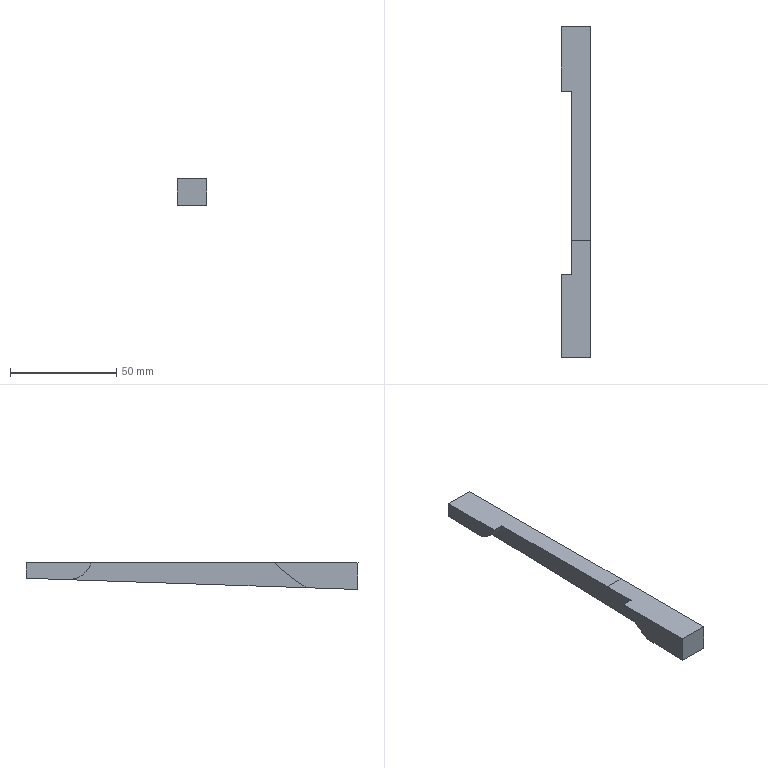Component | NX | UPPER_WEDGE | 1 solid | 11 faces | box 14 x 156.34 x 12.64 mm | volume 17054 mm3 | plane 9 | cylinder 2 | commonest cylinder face diameters 22.759 x1 150 x1
STEP:
#1=CARTESIAN_POINT('',(0.,0.,0.));
#2=DIRECTION('',(0.,0.,1.));
#3=DIRECTION('',(1.,0.,0.));
#4=AXIS2_PLACEMENT_3D('',#1,#2,#3);
#5=CARTESIAN_POINT('',(-109.,42.593,69.43));
#6=VERTEX_POINT('',#5);
#7=CARTESIAN_POINT('',(-109.,53.838,61.449));
#8=VERTEX_POINT('',#7);
#9=CARTESIAN_POINT('',(-109.,53.456,72.821));
#10=DIRECTION('',(1.,0.,0.));
#11=DIRECTION('',(0.,1.,-0.0009895));
#12=AXIS2_PLACEMENT_3D('',#9,#10,#11);
#13=CIRCLE('',#12,11.379);
#14=CARTESIAN_POINT('',(-109.,73.093,69.4));
#15=DIRECTION('',(-1.,0.,0.));
#16=DIRECTION('',(0.,0.03361,-0.9994));
#17=AXIS2_PLACEMENT_3D('',#14,#15,#16);
#18=PLANE('',#17);
#19=CARTESIAN_POINT('',(-3.686,8.139));
#20=CARTESIAN_POINT('',(-23.383,7.457));
#21=CARTESIAN_POINT('',(-14.125,24.857));
#22=CARTESIAN_POINT('',(-4.867,42.257));
#23=CARTESIAN_POINT('',(5.573,25.539));
#24=CARTESIAN_POINT('',(16.012,8.821));
#25=CARTESIAN_POINT('',(-3.686,8.139));
#26=(BOUNDED_CURVE()B_SPLINE_CURVE(2,(#19,#20,#21,#22,#23,#24,#25),.UNSPECIFIED.,.T.,.F.)B_SPLINE_CURVE_WITH_KNOTS((1,2,2,2,2,1),(-2.094,0.,2.094,4.189,6.283,8.378),.UNSPECIFIED.)CURVE()GEOMETRIC_REPRESENTATION_ITEM()RATIONAL_B_SPLINE_CURVE((1.,0.5,1.,0.5,1.,0.5,1.))REPRESENTATION_ITEM(''));
#27=(GEOMETRIC_REPRESENTATION_CONTEXT(2)PARAMETRIC_REPRESENTATION_CONTEXT()REPRESENTATION_CONTEXT('',''));
#28=DEFINITIONAL_REPRESENTATION('',(#26),#27);
#29=PCURVE('',#18,#28);
#30=CARTESIAN_POINT('',(-104.,53.456,72.821));
#31=DIRECTION('',(-1.,0.,0.));
#32=DIRECTION('',(0.,0.03361,-0.9994));
#33=AXIS2_PLACEMENT_3D('',#30,#31,#32);
#34=CYLINDRICAL_SURFACE('',#33,11.379);
#35=CARTESIAN_POINT('',(4.747,5.));
#36=DIRECTION('',(-1.,0.));
#37=VECTOR('',#36,1.);
#38=LINE('',#35,#37);
#39=(GEOMETRIC_REPRESENTATION_CONTEXT(2)PARAMETRIC_REPRESENTATION_CONTEXT()REPRESENTATION_CONTEXT('',''));
#40=DEFINITIONAL_REPRESENTATION('',(#38),#39);
#41=PCURVE('',#34,#40);
#42=SURFACE_CURVE('',#13,(#29,#41),.PCURVE_S1.);
#43=EDGE_CURVE('',#6,#8,#42,.T.);
#44=ORIENTED_EDGE('',*,*,#43,.F.);
#45=CARTESIAN_POINT('',(-109.,73.093,69.4));
#46=VERTEX_POINT('',#45);
#47=CARTESIAN_POINT('',(-109.,-83.,69.555));
#48=DIRECTION('',(0.,1.,-0.0009895));
#49=VECTOR('',#48,1.);
#50=LINE('',#47,#49);
#51=CARTESIAN_POINT('',(-5.4,156.));
#52=DIRECTION('',(0.03459,-0.9994));
#53=VECTOR('',#52,1.);
#54=LINE('',#51,#53);
#55=(GEOMETRIC_REPRESENTATION_CONTEXT(2)PARAMETRIC_REPRESENTATION_CONTEXT()REPRESENTATION_CONTEXT('',''));
#56=DEFINITIONAL_REPRESENTATION('',(#54),#55);
#57=PCURVE('',#18,#56);
#58=CARTESIAN_POINT('',(-95.,73.093,69.4));
#59=DIRECTION('',(0.,-0.0009895,-1.));
#60=DIRECTION('',(0.,1.,-0.0009895));
#61=AXIS2_PLACEMENT_3D('',#58,#59,#60);
#62=PLANE('',#61);
#63=CARTESIAN_POINT('',(-156.093,-14.));
#64=DIRECTION('',(1.,0.));
#65=VECTOR('',#64,1.);
#66=LINE('',#63,#65);
#67=(GEOMETRIC_REPRESENTATION_CONTEXT(2)PARAMETRIC_REPRESENTATION_CONTEXT()REPRESENTATION_CONTEXT('',''));
#68=DEFINITIONAL_REPRESENTATION('',(#66),#67);
#69=PCURVE('',#62,#68);
#70=SURFACE_CURVE('',#50,(#57,#69),.PCURVE_S1.);
#71=EDGE_CURVE('',#6,#46,#70,.T.);
#72=ORIENTED_EDGE('',*,*,#71,.T.);
#73=CARTESIAN_POINT('',(-109.,73.339,62.104));
#74=VERTEX_POINT('',#73);
#75=CARTESIAN_POINT('',(-109.,73.093,69.4));
#76=DIRECTION('',(0.,0.03361,-0.9994));
#77=VECTOR('',#76,1.);
#78=LINE('',#75,#77);
#79=CARTESIAN_POINT('',(0.,0.));
#80=DIRECTION('',(1.,0.));
#81=VECTOR('',#80,1.);
#82=LINE('',#79,#81);
#83=(GEOMETRIC_REPRESENTATION_CONTEXT(2)PARAMETRIC_REPRESENTATION_CONTEXT()REPRESENTATION_CONTEXT('',''));
#84=DEFINITIONAL_REPRESENTATION('',(#82),#83);
#85=PCURVE('',#18,#84);
#86=CARTESIAN_POINT('',(-95.,73.339,62.104));
#87=DIRECTION('',(0.,-0.9994,-0.03361));
#88=DIRECTION('',(0.,0.03361,-0.9994));
#89=AXIS2_PLACEMENT_3D('',#86,#87,#88);
#90=PLANE('',#89);
#91=CARTESIAN_POINT('',(-7.3,-14.));
#92=DIRECTION('',(1.,0.));
#93=VECTOR('',#92,1.);
#94=LINE('',#91,#93);
#95=(GEOMETRIC_REPRESENTATION_CONTEXT(2)PARAMETRIC_REPRESENTATION_CONTEXT()REPRESENTATION_CONTEXT('',''));
#96=DEFINITIONAL_REPRESENTATION('',(#94),#95);
#97=PCURVE('',#90,#96);
#98=SURFACE_CURVE('',#78,(#85,#97),.PCURVE_S1.);
#99=EDGE_CURVE('',#46,#74,#98,.T.);
#100=ORIENTED_EDGE('',*,*,#99,.T.);
#101=CARTESIAN_POINT('',(-109.,73.339,62.104));
#102=DIRECTION('',(0.,-0.9994,-0.03361));
#103=VECTOR('',#102,1.);
#104=LINE('',#101,#103);
#105=CARTESIAN_POINT('',(7.3,-0.));
#106=DIRECTION('',(-0.,1.));
#107=VECTOR('',#106,1.);
#108=LINE('',#105,#107);
#109=(GEOMETRIC_REPRESENTATION_CONTEXT(2)PARAMETRIC_REPRESENTATION_CONTEXT()REPRESENTATION_CONTEXT('',''));
#110=DEFINITIONAL_REPRESENTATION('',(#108),#109);
#111=PCURVE('',#18,#110);
#112=CARTESIAN_POINT('',(-95.,-82.573,56.862));
#113=DIRECTION('',(0.,-0.03361,0.9994));
#114=DIRECTION('',(-1.,0.,0.));
#115=AXIS2_PLACEMENT_3D('',#112,#113,#114);
#116=PLANE('',#115);
#117=CARTESIAN_POINT('',(14.,-156.));
#118=DIRECTION('',(0.,1.));
#119=VECTOR('',#118,1.);
#120=LINE('',#117,#119);
#121=(GEOMETRIC_REPRESENTATION_CONTEXT(2)PARAMETRIC_REPRESENTATION_CONTEXT()REPRESENTATION_CONTEXT('',''));
#122=DEFINITIONAL_REPRESENTATION('',(#120),#121);
#123=PCURVE('',#116,#122);
#124=SURFACE_CURVE('',#104,(#111,#123),.PCURVE_S1.);
#125=EDGE_CURVE('',#74,#8,#124,.T.);
#126=ORIENTED_EDGE('',*,*,#125,.T.);
#127=EDGE_LOOP('',(#44,#72,#100,#126));
#128=FACE_BOUND('',#127,.T.);
#129=ADVANCED_FACE('',(#128),#18,.T.);
#130=CARTESIAN_POINT('',(-109.,-43.516,69.5));
#131=VERTEX_POINT('',#130);
#132=CARTESIAN_POINT('',(-109.,-82.998,69.5));
#133=VERTEX_POINT('',#132);
#134=CARTESIAN_POINT('',(-109.,73.093,69.5));
#135=DIRECTION('',(0.,-1.,0.));
#136=VECTOR('',#135,1.);
#137=LINE('',#134,#136);
#138=CARTESIAN_POINT('',(-109.,73.093,69.4));
#139=DIRECTION('',(-1.,0.,0.));
#140=DIRECTION('',(0.,0.03361,-0.9994));
#141=AXIS2_PLACEMENT_3D('',#138,#139,#140);
#142=PLANE('',#141);
#143=CARTESIAN_POINT('',(-0.09982,-0.003356));
#144=DIRECTION('',(-0.03361,0.9994));
#145=VECTOR('',#144,1.);
#146=LINE('',#143,#145);
#147=(GEOMETRIC_REPRESENTATION_CONTEXT(2)PARAMETRIC_REPRESENTATION_CONTEXT()REPRESENTATION_CONTEXT('',''));
#148=DEFINITIONAL_REPRESENTATION('',(#146),#147);
#149=PCURVE('',#142,#148);
#150=CARTESIAN_POINT('',(-100.,0.,69.5));
#151=DIRECTION('',(0.,0.,-1.));
#152=DIRECTION('',(-1.,0.,0.));
#153=AXIS2_PLACEMENT_3D('',#150,#151,#152);
#154=PLANE('',#153);
#155=CARTESIAN_POINT('',(9.,73.093));
#156=DIRECTION('',(0.,-1.));
#157=VECTOR('',#156,1.);
#158=LINE('',#155,#157);
#159=(GEOMETRIC_REPRESENTATION_CONTEXT(2)PARAMETRIC_REPRESENTATION_CONTEXT()REPRESENTATION_CONTEXT('',''));
#160=DEFINITIONAL_REPRESENTATION('',(#158),#159);
#161=PCURVE('',#154,#160);
#162=SURFACE_CURVE('',#137,(#149,#161),.PCURVE_S1.);
#163=EDGE_CURVE('',#131,#133,#162,.T.);
#164=ORIENTED_EDGE('',*,*,#163,.F.);
#165=CARTESIAN_POINT('',(-109.,-59.072,57.652));
#166=VERTEX_POINT('',#165);
#167=CARTESIAN_POINT('',(-109.,-96.348,122.733));
#168=DIRECTION('',(1.,0.,0.));
#169=DIRECTION('',(0.,1.,-0.0009895));
#170=AXIS2_PLACEMENT_3D('',#167,#168,#169);
#171=CIRCLE('',#170,75.);
#172=CARTESIAN_POINT('',(-56.402,92.598));
#173=CARTESIAN_POINT('',(-186.228,88.104));
#174=CARTESIAN_POINT('',(-125.207,202.784));
#175=CARTESIAN_POINT('',(-64.186,317.464));
#176=CARTESIAN_POINT('',(4.619,207.278));
#177=CARTESIAN_POINT('',(73.424,97.092));
#178=CARTESIAN_POINT('',(-56.402,92.598));
#179=(BOUNDED_CURVE()B_SPLINE_CURVE(2,(#172,#173,#174,#175,#176,#177,#178),.UNSPECIFIED.,.T.,.F.)B_SPLINE_CURVE_WITH_KNOTS((1,2,2,2,2,1),(-2.094,0.,2.094,4.189,6.283,8.378),.UNSPECIFIED.)CURVE()GEOMETRIC_REPRESENTATION_ITEM()RATIONAL_B_SPLINE_CURVE((1.,0.5,1.,0.5,1.,0.5,1.))REPRESENTATION_ITEM(''));
#180=(GEOMETRIC_REPRESENTATION_CONTEXT(2)PARAMETRIC_REPRESENTATION_CONTEXT()REPRESENTATION_CONTEXT('',''));
#181=DEFINITIONAL_REPRESENTATION('',(#179),#180);
#182=PCURVE('',#142,#181);
#183=CARTESIAN_POINT('',(-104.,-96.348,122.733));
#184=DIRECTION('',(-1.,0.,0.));
#185=DIRECTION('',(0.,0.03361,-0.9994));
#186=AXIS2_PLACEMENT_3D('',#183,#184,#185);
#187=CYLINDRICAL_SURFACE('',#186,75.);
#188=CARTESIAN_POINT('',(11.03,5.));
#189=DIRECTION('',(-1.,0.));
#190=VECTOR('',#189,1.);
#191=LINE('',#188,#190);
#192=(GEOMETRIC_REPRESENTATION_CONTEXT(2)PARAMETRIC_REPRESENTATION_CONTEXT()REPRESENTATION_CONTEXT('',''));
#193=DEFINITIONAL_REPRESENTATION('',(#191),#192);
#194=PCURVE('',#187,#193);
#195=SURFACE_CURVE('',#171,(#182,#194),.PCURVE_S1.);
#196=EDGE_CURVE('',#166,#131,#195,.T.);
#197=ORIENTED_EDGE('',*,*,#196,.F.);
#198=CARTESIAN_POINT('',(-109.,-82.573,56.862));
#199=VERTEX_POINT('',#198);
#200=CARTESIAN_POINT('',(-109.,73.339,62.104));
#201=DIRECTION('',(0.,-0.9994,-0.03361));
#202=VECTOR('',#201,1.);
#203=LINE('',#200,#202);
#204=CARTESIAN_POINT('',(7.3,-0.));
#205=DIRECTION('',(-0.,1.));
#206=VECTOR('',#205,1.);
#207=LINE('',#204,#206);
#208=(GEOMETRIC_REPRESENTATION_CONTEXT(2)PARAMETRIC_REPRESENTATION_CONTEXT()REPRESENTATION_CONTEXT('',''));
#209=DEFINITIONAL_REPRESENTATION('',(#207),#208);
#210=PCURVE('',#142,#209);
#211=CARTESIAN_POINT('',(14.,-156.));
#212=DIRECTION('',(0.,1.));
#213=VECTOR('',#212,1.);
#214=LINE('',#211,#213);
#215=(GEOMETRIC_REPRESENTATION_CONTEXT(2)PARAMETRIC_REPRESENTATION_CONTEXT()REPRESENTATION_CONTEXT('',''));
#216=DEFINITIONAL_REPRESENTATION('',(#214),#215);
#217=PCURVE('',#116,#216);
#218=SURFACE_CURVE('',#203,(#210,#217),.PCURVE_S1.);
#219=EDGE_CURVE('',#166,#199,#218,.T.);
#220=ORIENTED_EDGE('',*,*,#219,.T.);
#221=CARTESIAN_POINT('',(-109.,-82.573,56.862));
#222=DIRECTION('',(0.,-0.03361,0.9994));
#223=VECTOR('',#222,1.);
#224=LINE('',#221,#223);
#225=CARTESIAN_POINT('',(7.3,156.));
#226=DIRECTION('',(-1.,0.));
#227=VECTOR('',#226,1.);
#228=LINE('',#225,#227);
#229=(GEOMETRIC_REPRESENTATION_CONTEXT(2)PARAMETRIC_REPRESENTATION_CONTEXT()REPRESENTATION_CONTEXT('',''));
#230=DEFINITIONAL_REPRESENTATION('',(#228),#229);
#231=PCURVE('',#142,#230);
#232=CARTESIAN_POINT('',(-95.,-83.,69.555));
#233=DIRECTION('',(0.,0.9994,0.03361));
#234=DIRECTION('',(0.,-0.03361,0.9994));
#235=AXIS2_PLACEMENT_3D('',#232,#233,#234);
#236=PLANE('',#235);
#237=CARTESIAN_POINT('',(-12.7,-14.));
#238=DIRECTION('',(1.,0.));
#239=VECTOR('',#238,1.);
#240=LINE('',#237,#239);
#241=(GEOMETRIC_REPRESENTATION_CONTEXT(2)PARAMETRIC_REPRESENTATION_CONTEXT()REPRESENTATION_CONTEXT('',''));
#242=DEFINITIONAL_REPRESENTATION('',(#240),#241);
#243=PCURVE('',#236,#242);
#244=SURFACE_CURVE('',#224,(#231,#243),.PCURVE_S1.);
#245=EDGE_CURVE('',#199,#133,#244,.T.);
#246=ORIENTED_EDGE('',*,*,#245,.T.);
#247=EDGE_LOOP('',(#164,#197,#220,#246));
#248=FACE_BOUND('',#247,.T.);
#249=ADVANCED_FACE('',(#248),#142,.T.);
#250=ORIENTED_EDGE('',*,*,#99,.F.);
#251=CARTESIAN_POINT('',(-95.,73.093,69.4));
#252=VERTEX_POINT('',#251);
#253=CARTESIAN_POINT('',(-95.,73.093,69.4));
#254=DIRECTION('',(-1.,0.,0.));
#255=VECTOR('',#254,1.);
#256=LINE('',#253,#255);
#257=CARTESIAN_POINT('',(-7.3,0.));
#258=DIRECTION('',(0.,-1.));
#259=VECTOR('',#258,1.);
#260=LINE('',#257,#259);
#261=(GEOMETRIC_REPRESENTATION_CONTEXT(2)PARAMETRIC_REPRESENTATION_CONTEXT()REPRESENTATION_CONTEXT('',''));
#262=DEFINITIONAL_REPRESENTATION('',(#260),#261);
#263=PCURVE('',#90,#262);
#264=CARTESIAN_POINT('',(0.,0.));
#265=DIRECTION('',(0.,-1.));
#266=VECTOR('',#265,1.);
#267=LINE('',#264,#266);
#268=(GEOMETRIC_REPRESENTATION_CONTEXT(2)PARAMETRIC_REPRESENTATION_CONTEXT()REPRESENTATION_CONTEXT('',''));
#269=DEFINITIONAL_REPRESENTATION('',(#267),#268);
#270=PCURVE('',#62,#269);
#271=SURFACE_CURVE('',#256,(#263,#270),.PCURVE_S1.);
#272=EDGE_CURVE('',#252,#46,#271,.T.);
#273=ORIENTED_EDGE('',*,*,#272,.F.);
#274=CARTESIAN_POINT('',(-95.,73.339,62.104));
#275=VERTEX_POINT('',#274);
#276=CARTESIAN_POINT('',(-95.,73.339,62.104));
#277=DIRECTION('',(0.,-0.03361,0.9994));
#278=VECTOR('',#277,1.);
#279=LINE('',#276,#278);
#280=CARTESIAN_POINT('',(0.,0.));
#281=DIRECTION('',(-1.,0.));
#282=VECTOR('',#281,1.);
#283=LINE('',#280,#282);
#284=(GEOMETRIC_REPRESENTATION_CONTEXT(2)PARAMETRIC_REPRESENTATION_CONTEXT()REPRESENTATION_CONTEXT('',''));
#285=DEFINITIONAL_REPRESENTATION('',(#283),#284);
#286=PCURVE('',#90,#285);
#287=CARTESIAN_POINT('',(-95.,73.093,69.4));
#288=DIRECTION('',(-1.,0.,0.));
#289=DIRECTION('',(0.,0.03361,-0.9994));
#290=AXIS2_PLACEMENT_3D('',#287,#288,#289);
#291=PLANE('',#290);
#292=CARTESIAN_POINT('',(7.3,-0.));
#293=DIRECTION('',(-1.,0.));
#294=VECTOR('',#293,1.);
#295=LINE('',#292,#294);
#296=(GEOMETRIC_REPRESENTATION_CONTEXT(2)PARAMETRIC_REPRESENTATION_CONTEXT()REPRESENTATION_CONTEXT('',''));
#297=DEFINITIONAL_REPRESENTATION('',(#295),#296);
#298=PCURVE('',#291,#297);
#299=SURFACE_CURVE('',#279,(#286,#298),.PCURVE_S1.);
#300=EDGE_CURVE('',#275,#252,#299,.T.);
#301=ORIENTED_EDGE('',*,*,#300,.F.);
#302=CARTESIAN_POINT('',(-95.,73.339,62.104));
#303=DIRECTION('',(-1.,0.,0.));
#304=VECTOR('',#303,1.);
#305=LINE('',#302,#304);
#306=CARTESIAN_POINT('',(0.,0.));
#307=DIRECTION('',(0.,-1.));
#308=VECTOR('',#307,1.);
#309=LINE('',#306,#308);
#310=(GEOMETRIC_REPRESENTATION_CONTEXT(2)PARAMETRIC_REPRESENTATION_CONTEXT()REPRESENTATION_CONTEXT('',''));
#311=DEFINITIONAL_REPRESENTATION('',(#309),#310);
#312=PCURVE('',#90,#311);
#313=CARTESIAN_POINT('',(0.,-156.));
#314=DIRECTION('',(1.,0.));
#315=VECTOR('',#314,1.);
#316=LINE('',#313,#315);
#317=(GEOMETRIC_REPRESENTATION_CONTEXT(2)PARAMETRIC_REPRESENTATION_CONTEXT()REPRESENTATION_CONTEXT('',''));
#318=DEFINITIONAL_REPRESENTATION('',(#316),#317);
#319=PCURVE('',#116,#318);
#320=SURFACE_CURVE('',#305,(#312,#319),.PCURVE_S1.);
#321=EDGE_CURVE('',#275,#74,#320,.T.);
#322=ORIENTED_EDGE('',*,*,#321,.T.);
#323=EDGE_LOOP('',(#250,#273,#301,#322));
#324=FACE_BOUND('',#323,.T.);
#325=ADVANCED_FACE('',(#324),#90,.F.);
#326=CARTESIAN_POINT('',(-104.,-27.834,69.5));
#327=VERTEX_POINT('',#326);
#328=CARTESIAN_POINT('',(-104.,42.593,69.43));
#329=VERTEX_POINT('',#328);
#330=CARTESIAN_POINT('',(-104.,-43.5,69.516));
#331=DIRECTION('',(0.,1.,-0.0009895));
#332=VECTOR('',#331,1.);
#333=LINE('',#330,#332);
#334=CARTESIAN_POINT('',(-116.593,-9.));
#335=DIRECTION('',(1.,0.));
#336=VECTOR('',#335,1.);
#337=LINE('',#334,#336);
#338=(GEOMETRIC_REPRESENTATION_CONTEXT(2)PARAMETRIC_REPRESENTATION_CONTEXT()REPRESENTATION_CONTEXT('',''));
#339=DEFINITIONAL_REPRESENTATION('',(#337),#338);
#340=PCURVE('',#62,#339);
#341=CARTESIAN_POINT('',(-104.,53.456,72.821));
#342=DIRECTION('',(1.,0.,0.));
#343=DIRECTION('',(0.,-0.03361,0.9994));
#344=AXIS2_PLACEMENT_3D('',#341,#342,#343);
#345=PLANE('',#344);
#346=CARTESIAN_POINT('',(-0.04575,97.012));
#347=DIRECTION('',(-0.03459,-0.9994));
#348=VECTOR('',#347,1.);
#349=LINE('',#346,#348);
#350=(GEOMETRIC_REPRESENTATION_CONTEXT(2)PARAMETRIC_REPRESENTATION_CONTEXT()REPRESENTATION_CONTEXT('',''));
#351=DEFINITIONAL_REPRESENTATION('',(#349),#350);
#352=PCURVE('',#345,#351);
#353=SURFACE_CURVE('',#333,(#340,#352),.PCURVE_S1.);
#354=EDGE_CURVE('',#327,#329,#353,.T.);
#355=ORIENTED_EDGE('',*,*,#354,.F.);
#356=CARTESIAN_POINT('',(-95.,-27.834,69.5));
#357=VERTEX_POINT('',#356);
#358=CARTESIAN_POINT('',(-95.,-27.834,69.5));
#359=DIRECTION('',(1.,0.,0.));
#360=VECTOR('',#359,1.);
#361=LINE('',#358,#360);
#362=CARTESIAN_POINT('',(-100.928,0.));
#363=DIRECTION('',(0.,1.));
#364=VECTOR('',#363,1.);
#365=LINE('',#362,#364);
#366=(GEOMETRIC_REPRESENTATION_CONTEXT(2)PARAMETRIC_REPRESENTATION_CONTEXT()REPRESENTATION_CONTEXT('',''));
#367=DEFINITIONAL_REPRESENTATION('',(#365),#366);
#368=PCURVE('',#62,#367);
#369=CARTESIAN_POINT('',(-5.,-27.834));
#370=DIRECTION('',(-1.,0.));
#371=VECTOR('',#370,1.);
#372=LINE('',#369,#371);
#373=(GEOMETRIC_REPRESENTATION_CONTEXT(2)PARAMETRIC_REPRESENTATION_CONTEXT()REPRESENTATION_CONTEXT('',''));
#374=DEFINITIONAL_REPRESENTATION('',(#372),#373);
#375=PCURVE('',#154,#374);
#376=SURFACE_CURVE('',#361,(#368,#375),.PCURVE_S1.);
#377=EDGE_CURVE('',#327,#357,#376,.T.);
#378=ORIENTED_EDGE('',*,*,#377,.T.);
#379=CARTESIAN_POINT('',(-95.,73.093,69.4));
#380=DIRECTION('',(0.,-1.,0.0009895));
#381=VECTOR('',#380,1.);
#382=LINE('',#379,#381);
#383=CARTESIAN_POINT('',(0.,0.));
#384=DIRECTION('',(-1.,0.));
#385=VECTOR('',#384,1.);
#386=LINE('',#383,#385);
#387=(GEOMETRIC_REPRESENTATION_CONTEXT(2)PARAMETRIC_REPRESENTATION_CONTEXT()REPRESENTATION_CONTEXT('',''));
#388=DEFINITIONAL_REPRESENTATION('',(#386),#387);
#389=PCURVE('',#62,#388);
#390=CARTESIAN_POINT('',(0.,0.));
#391=DIRECTION('',(-0.03459,0.9994));
#392=VECTOR('',#391,1.);
#393=LINE('',#390,#392);
#394=(GEOMETRIC_REPRESENTATION_CONTEXT(2)PARAMETRIC_REPRESENTATION_CONTEXT()REPRESENTATION_CONTEXT('',''));
#395=DEFINITIONAL_REPRESENTATION('',(#393),#394);
#396=PCURVE('',#291,#395);
#397=SURFACE_CURVE('',#382,(#389,#396),.PCURVE_S1.);
#398=EDGE_CURVE('',#252,#357,#397,.T.);
#399=ORIENTED_EDGE('',*,*,#398,.F.);
#400=ORIENTED_EDGE('',*,*,#272,.T.);
#401=ORIENTED_EDGE('',*,*,#71,.F.);
#402=CARTESIAN_POINT('',(-104.,42.593,69.43));
#403=DIRECTION('',(-1.,0.,0.));
#404=VECTOR('',#403,1.);
#405=LINE('',#402,#404);
#406=CARTESIAN_POINT('',(-30.5,-9.));
#407=DIRECTION('',(0.,-1.));
#408=VECTOR('',#407,1.);
#409=LINE('',#406,#408);
#410=(GEOMETRIC_REPRESENTATION_CONTEXT(2)PARAMETRIC_REPRESENTATION_CONTEXT()REPRESENTATION_CONTEXT('',''));
#411=DEFINITIONAL_REPRESENTATION('',(#409),#410);
#412=PCURVE('',#62,#411);
#413=CARTESIAN_POINT('',(1.302,0.));
#414=DIRECTION('',(0.,1.));
#415=VECTOR('',#414,1.);
#416=LINE('',#413,#415);
#417=(GEOMETRIC_REPRESENTATION_CONTEXT(2)PARAMETRIC_REPRESENTATION_CONTEXT()REPRESENTATION_CONTEXT('',''));
#418=DEFINITIONAL_REPRESENTATION('',(#416),#417);
#419=PCURVE('',#34,#418);
#420=SURFACE_CURVE('',#405,(#412,#419),.PCURVE_S1.);
#421=EDGE_CURVE('',#329,#6,#420,.T.);
#422=ORIENTED_EDGE('',*,*,#421,.F.);
#423=EDGE_LOOP('',(#355,#378,#399,#400,#401,#422));
#424=FACE_BOUND('',#423,.T.);
#425=ADVANCED_FACE('',(#424),#62,.F.);
#426=CARTESIAN_POINT('',(-95.,-82.998,69.5));
#427=VERTEX_POINT('',#426);
#428=CARTESIAN_POINT('',(-95.,-82.573,56.862));
#429=VERTEX_POINT('',#428);
#430=CARTESIAN_POINT('',(-95.,-83.,69.555));
#431=DIRECTION('',(0.,0.03361,-0.9994));
#432=VECTOR('',#431,1.);
#433=LINE('',#430,#432);
#434=CARTESIAN_POINT('',(0.,0.));
#435=DIRECTION('',(-1.,0.));
#436=VECTOR('',#435,1.);
#437=LINE('',#434,#436);
#438=(GEOMETRIC_REPRESENTATION_CONTEXT(2)PARAMETRIC_REPRESENTATION_CONTEXT()REPRESENTATION_CONTEXT('',''));
#439=DEFINITIONAL_REPRESENTATION('',(#437),#438);
#440=PCURVE('',#236,#439);
#441=CARTESIAN_POINT('',(-5.4,156.));
#442=DIRECTION('',(1.,0.));
#443=VECTOR('',#442,1.);
#444=LINE('',#441,#443);
#445=(GEOMETRIC_REPRESENTATION_CONTEXT(2)PARAMETRIC_REPRESENTATION_CONTEXT()REPRESENTATION_CONTEXT('',''));
#446=DEFINITIONAL_REPRESENTATION('',(#444),#445);
#447=PCURVE('',#291,#446);
#448=SURFACE_CURVE('',#433,(#440,#447),.PCURVE_S1.);
#449=EDGE_CURVE('',#427,#429,#448,.T.);
#450=ORIENTED_EDGE('',*,*,#449,.F.);
#451=CARTESIAN_POINT('',(-95.,-82.998,69.5));
#452=DIRECTION('',(-1.,0.,0.));
#453=VECTOR('',#452,1.);
#454=LINE('',#451,#453);
#455=CARTESIAN_POINT('',(-0.05462,0.));
#456=DIRECTION('',(0.,-1.));
#457=VECTOR('',#456,1.);
#458=LINE('',#455,#457);
#459=(GEOMETRIC_REPRESENTATION_CONTEXT(2)PARAMETRIC_REPRESENTATION_CONTEXT()REPRESENTATION_CONTEXT('',''));
#460=DEFINITIONAL_REPRESENTATION('',(#458),#459);
#461=PCURVE('',#236,#460);
#462=CARTESIAN_POINT('',(-5.,-82.998));
#463=DIRECTION('',(1.,0.));
#464=VECTOR('',#463,1.);
#465=LINE('',#462,#464);
#466=(GEOMETRIC_REPRESENTATION_CONTEXT(2)PARAMETRIC_REPRESENTATION_CONTEXT()REPRESENTATION_CONTEXT('',''));
#467=DEFINITIONAL_REPRESENTATION('',(#465),#466);
#468=PCURVE('',#154,#467);
#469=SURFACE_CURVE('',#454,(#461,#468),.PCURVE_S1.);
#470=EDGE_CURVE('',#427,#133,#469,.T.);
#471=ORIENTED_EDGE('',*,*,#470,.T.);
#472=ORIENTED_EDGE('',*,*,#245,.F.);
#473=CARTESIAN_POINT('',(-95.,-82.573,56.862));
#474=DIRECTION('',(-1.,0.,0.));
#475=VECTOR('',#474,1.);
#476=LINE('',#473,#475);
#477=CARTESIAN_POINT('',(-12.7,0.));
#478=DIRECTION('',(0.,-1.));
#479=VECTOR('',#478,1.);
#480=LINE('',#477,#479);
#481=(GEOMETRIC_REPRESENTATION_CONTEXT(2)PARAMETRIC_REPRESENTATION_CONTEXT()REPRESENTATION_CONTEXT('',''));
#482=DEFINITIONAL_REPRESENTATION('',(#480),#481);
#483=PCURVE('',#236,#482);
#484=CARTESIAN_POINT('',(0.,0.));
#485=DIRECTION('',(1.,0.));
#486=VECTOR('',#485,1.);
#487=LINE('',#484,#486);
#488=(GEOMETRIC_REPRESENTATION_CONTEXT(2)PARAMETRIC_REPRESENTATION_CONTEXT()REPRESENTATION_CONTEXT('',''));
#489=DEFINITIONAL_REPRESENTATION('',(#487),#488);
#490=PCURVE('',#116,#489);
#491=SURFACE_CURVE('',#476,(#483,#490),.PCURVE_S1.);
#492=EDGE_CURVE('',#429,#199,#491,.T.);
#493=ORIENTED_EDGE('',*,*,#492,.F.);
#494=EDGE_LOOP('',(#450,#471,#472,#493));
#495=FACE_BOUND('',#494,.T.);
#496=ADVANCED_FACE('',(#495),#236,.F.);
#497=CARTESIAN_POINT('',(-104.,53.838,61.449));
#498=VERTEX_POINT('',#497);
#499=CARTESIAN_POINT('',(-104.,-59.072,57.652));
#500=VERTEX_POINT('',#499);
#501=CARTESIAN_POINT('',(-104.,53.838,61.449));
#502=DIRECTION('',(0.,-0.9994,-0.03361));
#503=VECTOR('',#502,1.);
#504=LINE('',#501,#503);
#505=CARTESIAN_POINT('',(9.,-136.488));
#506=DIRECTION('',(0.,1.));
#507=VECTOR('',#506,1.);
#508=LINE('',#505,#507);
#509=(GEOMETRIC_REPRESENTATION_CONTEXT(2)PARAMETRIC_REPRESENTATION_CONTEXT()REPRESENTATION_CONTEXT('',''));
#510=DEFINITIONAL_REPRESENTATION('',(#508),#509);
#511=PCURVE('',#116,#510);
#512=CARTESIAN_POINT('',(-11.379,0.));
#513=DIRECTION('',(0.,1.));
#514=VECTOR('',#513,1.);
#515=LINE('',#512,#514);
#516=(GEOMETRIC_REPRESENTATION_CONTEXT(2)PARAMETRIC_REPRESENTATION_CONTEXT()REPRESENTATION_CONTEXT('',''));
#517=DEFINITIONAL_REPRESENTATION('',(#515),#516);
#518=PCURVE('',#345,#517);
#519=SURFACE_CURVE('',#504,(#511,#518),.PCURVE_S1.);
#520=EDGE_CURVE('',#498,#500,#519,.T.);
#521=ORIENTED_EDGE('',*,*,#520,.F.);
#522=CARTESIAN_POINT('',(-104.,53.838,61.449));
#523=DIRECTION('',(-1.,0.,0.));
#524=VECTOR('',#523,1.);
#525=LINE('',#522,#524);
#526=CARTESIAN_POINT('',(9.,-136.488));
#527=DIRECTION('',(1.,0.));
#528=VECTOR('',#527,1.);
#529=LINE('',#526,#528);
#530=(GEOMETRIC_REPRESENTATION_CONTEXT(2)PARAMETRIC_REPRESENTATION_CONTEXT()REPRESENTATION_CONTEXT('',''));
#531=DEFINITIONAL_REPRESENTATION('',(#529),#530);
#532=PCURVE('',#116,#531);
#533=CARTESIAN_POINT('',(0.,0.));
#534=DIRECTION('',(0.,1.));
#535=VECTOR('',#534,1.);
#536=LINE('',#533,#535);
#537=(GEOMETRIC_REPRESENTATION_CONTEXT(2)PARAMETRIC_REPRESENTATION_CONTEXT()REPRESENTATION_CONTEXT('',''));
#538=DEFINITIONAL_REPRESENTATION('',(#536),#537);
#539=PCURVE('',#34,#538);
#540=SURFACE_CURVE('',#525,(#532,#539),.PCURVE_S1.);
#541=EDGE_CURVE('',#498,#8,#540,.T.);
#542=ORIENTED_EDGE('',*,*,#541,.T.);
#543=ORIENTED_EDGE('',*,*,#125,.F.);
#544=ORIENTED_EDGE('',*,*,#321,.F.);
#545=CARTESIAN_POINT('',(-95.,-82.573,56.862));
#546=DIRECTION('',(0.,0.9994,0.03361));
#547=VECTOR('',#546,1.);
#548=LINE('',#545,#547);
#549=CARTESIAN_POINT('',(0.,0.));
#550=DIRECTION('',(0.,-1.));
#551=VECTOR('',#550,1.);
#552=LINE('',#549,#551);
#553=(GEOMETRIC_REPRESENTATION_CONTEXT(2)PARAMETRIC_REPRESENTATION_CONTEXT()REPRESENTATION_CONTEXT('',''));
#554=DEFINITIONAL_REPRESENTATION('',(#552),#553);
#555=PCURVE('',#116,#554);
#556=CARTESIAN_POINT('',(7.3,156.));
#557=DIRECTION('',(0.,-1.));
#558=VECTOR('',#557,1.);
#559=LINE('',#556,#558);
#560=(GEOMETRIC_REPRESENTATION_CONTEXT(2)PARAMETRIC_REPRESENTATION_CONTEXT()REPRESENTATION_CONTEXT('',''));
#561=DEFINITIONAL_REPRESENTATION('',(#559),#560);
#562=PCURVE('',#291,#561);
#563=SURFACE_CURVE('',#548,(#555,#562),.PCURVE_S1.);
#564=EDGE_CURVE('',#429,#275,#563,.T.);
#565=ORIENTED_EDGE('',*,*,#564,.F.);
#566=ORIENTED_EDGE('',*,*,#492,.T.);
#567=ORIENTED_EDGE('',*,*,#219,.F.);
#568=CARTESIAN_POINT('',(-104.,-59.072,57.652));
#569=DIRECTION('',(-1.,0.,0.));
#570=VECTOR('',#569,1.);
#571=LINE('',#568,#570);
#572=CARTESIAN_POINT('',(9.,-23.514));
#573=DIRECTION('',(1.,0.));
#574=VECTOR('',#573,1.);
#575=LINE('',#572,#574);
#576=(GEOMETRIC_REPRESENTATION_CONTEXT(2)PARAMETRIC_REPRESENTATION_CONTEXT()REPRESENTATION_CONTEXT('',''));
#577=DEFINITIONAL_REPRESENTATION('',(#575),#576);
#578=PCURVE('',#116,#577);
#579=CARTESIAN_POINT('',(5.797,0.));
#580=DIRECTION('',(0.,1.));
#581=VECTOR('',#580,1.);
#582=LINE('',#579,#581);
#583=(GEOMETRIC_REPRESENTATION_CONTEXT(2)PARAMETRIC_REPRESENTATION_CONTEXT()REPRESENTATION_CONTEXT('',''));
#584=DEFINITIONAL_REPRESENTATION('',(#582),#583);
#585=PCURVE('',#187,#584);
#586=SURFACE_CURVE('',#571,(#578,#585),.PCURVE_S1.);
#587=EDGE_CURVE('',#500,#166,#586,.T.);
#588=ORIENTED_EDGE('',*,*,#587,.F.);
#589=EDGE_LOOP('',(#521,#542,#543,#544,#565,#566,#567,#588));
#590=FACE_BOUND('',#589,.T.);
#591=ADVANCED_FACE('',(#590),#116,.F.);
#592=ORIENTED_EDGE('',*,*,#398,.T.);
#593=CARTESIAN_POINT('',(-95.,73.093,69.5));
#594=DIRECTION('',(0.,-1.,0.));
#595=VECTOR('',#594,1.);
#596=LINE('',#593,#595);
#597=CARTESIAN_POINT('',(-0.09982,-0.003356));
#598=DIRECTION('',(-0.03361,0.9994));
#599=VECTOR('',#598,1.);
#600=LINE('',#597,#599);
#601=(GEOMETRIC_REPRESENTATION_CONTEXT(2)PARAMETRIC_REPRESENTATION_CONTEXT()REPRESENTATION_CONTEXT('',''));
#602=DEFINITIONAL_REPRESENTATION('',(#600),#601);
#603=PCURVE('',#291,#602);
#604=CARTESIAN_POINT('',(-5.,73.093));
#605=DIRECTION('',(0.,-1.));
#606=VECTOR('',#605,1.);
#607=LINE('',#604,#606);
#608=(GEOMETRIC_REPRESENTATION_CONTEXT(2)PARAMETRIC_REPRESENTATION_CONTEXT()REPRESENTATION_CONTEXT('',''));
#609=DEFINITIONAL_REPRESENTATION('',(#607),#608);
#610=PCURVE('',#154,#609);
#611=SURFACE_CURVE('',#596,(#603,#610),.PCURVE_S1.);
#612=EDGE_CURVE('',#357,#427,#611,.T.);
#613=ORIENTED_EDGE('',*,*,#612,.T.);
#614=ORIENTED_EDGE('',*,*,#449,.T.);
#615=ORIENTED_EDGE('',*,*,#564,.T.);
#616=ORIENTED_EDGE('',*,*,#300,.T.);
#617=EDGE_LOOP('',(#592,#613,#614,#615,#616));
#618=FACE_BOUND('',#617,.T.);
#619=ADVANCED_FACE('',(#618),#291,.F.);
#620=ORIENTED_EDGE('',*,*,#43,.T.);
#621=ORIENTED_EDGE('',*,*,#541,.F.);
#622=CARTESIAN_POINT('',(-104.,53.456,72.821));
#623=DIRECTION('',(-1.,0.,0.));
#624=DIRECTION('',(0.,1.,-0.0009895));
#625=AXIS2_PLACEMENT_3D('',#622,#623,#624);
#626=CIRCLE('',#625,11.379);
#627=CARTESIAN_POINT('',(-1.536,0.));
#628=DIRECTION('',(1.,0.));
#629=VECTOR('',#628,1.);
#630=LINE('',#627,#629);
#631=(GEOMETRIC_REPRESENTATION_CONTEXT(2)PARAMETRIC_REPRESENTATION_CONTEXT()REPRESENTATION_CONTEXT('',''));
#632=DEFINITIONAL_REPRESENTATION('',(#630),#631);
#633=PCURVE('',#34,#632);
#634=CARTESIAN_POINT('',(-0.3937,-11.372));
#635=CARTESIAN_POINT('',(-20.091,-10.691));
#636=CARTESIAN_POINT('',(-9.652,6.027));
#637=CARTESIAN_POINT('',(0.7873,22.745));
#638=CARTESIAN_POINT('',(10.046,5.345));
#639=CARTESIAN_POINT('',(19.304,-12.054));
#640=CARTESIAN_POINT('',(-0.3937,-11.372));
#641=(BOUNDED_CURVE()B_SPLINE_CURVE(2,(#634,#635,#636,#637,#638,#639,#640),.UNSPECIFIED.,.T.,.F.)B_SPLINE_CURVE_WITH_KNOTS((1,2,2,2,2,1),(-2.094,0.,2.094,4.189,6.283,8.378),.UNSPECIFIED.)CURVE()GEOMETRIC_REPRESENTATION_ITEM()RATIONAL_B_SPLINE_CURVE((1.,0.5,1.,0.5,1.,0.5,1.))REPRESENTATION_ITEM(''));
#642=(GEOMETRIC_REPRESENTATION_CONTEXT(2)PARAMETRIC_REPRESENTATION_CONTEXT()REPRESENTATION_CONTEXT('',''));
#643=DEFINITIONAL_REPRESENTATION('',(#641),#642);
#644=PCURVE('',#345,#643);
#645=SURFACE_CURVE('',#626,(#633,#644),.PCURVE_S1.);
#646=EDGE_CURVE('',#498,#329,#645,.T.);
#647=ORIENTED_EDGE('',*,*,#646,.T.);
#648=ORIENTED_EDGE('',*,*,#421,.T.);
#649=EDGE_LOOP('',(#620,#621,#647,#648));
#650=FACE_BOUND('',#649,.T.);
#651=ADVANCED_FACE('',(#650),#34,.T.);
#652=ORIENTED_EDGE('',*,*,#196,.T.);
#653=CARTESIAN_POINT('',(-104.,-43.516,69.5));
#654=VERTEX_POINT('',#653);
#655=CARTESIAN_POINT('',(-104.,-43.516,69.5));
#656=DIRECTION('',(1.,0.,0.));
#657=VECTOR('',#656,1.);
#658=LINE('',#655,#657);
#659=CARTESIAN_POINT('',(5.535,0.));
#660=DIRECTION('',(0.,-1.));
#661=VECTOR('',#660,1.);
#662=LINE('',#659,#661);
#663=(GEOMETRIC_REPRESENTATION_CONTEXT(2)PARAMETRIC_REPRESENTATION_CONTEXT()REPRESENTATION_CONTEXT('',''));
#664=DEFINITIONAL_REPRESENTATION('',(#662),#663);
#665=PCURVE('',#187,#664);
#666=CARTESIAN_POINT('',(4.,-43.516));
#667=DIRECTION('',(-1.,0.));
#668=VECTOR('',#667,1.);
#669=LINE('',#666,#668);
#670=(GEOMETRIC_REPRESENTATION_CONTEXT(2)PARAMETRIC_REPRESENTATION_CONTEXT()REPRESENTATION_CONTEXT('',''));
#671=DEFINITIONAL_REPRESENTATION('',(#669),#670);
#672=PCURVE('',#154,#671);
#673=SURFACE_CURVE('',#658,(#665,#672),.PCURVE_S1.);
#674=EDGE_CURVE('',#131,#654,#673,.T.);
#675=ORIENTED_EDGE('',*,*,#674,.T.);
#676=CARTESIAN_POINT('',(-104.,-96.348,122.733));
#677=DIRECTION('',(-1.,0.,0.));
#678=DIRECTION('',(0.,1.,-0.0009895));
#679=AXIS2_PLACEMENT_3D('',#676,#677,#678);
#680=CIRCLE('',#679,75.);
#681=CARTESIAN_POINT('',(4.747,0.));
#682=DIRECTION('',(1.,0.));
#683=VECTOR('',#682,1.);
#684=LINE('',#681,#683);
#685=(GEOMETRIC_REPRESENTATION_CONTEXT(2)PARAMETRIC_REPRESENTATION_CONTEXT()REPRESENTATION_CONTEXT('',''));
#686=DEFINITIONAL_REPRESENTATION('',(#684),#685);
#687=PCURVE('',#187,#686);
#688=CARTESIAN_POINT('',(52.323,73.087));
#689=CARTESIAN_POINT('',(-77.503,77.58));
#690=CARTESIAN_POINT('',(-8.698,187.766));
#691=CARTESIAN_POINT('',(60.107,297.952));
#692=CARTESIAN_POINT('',(121.128,183.272));
#693=CARTESIAN_POINT('',(182.149,68.593));
#694=CARTESIAN_POINT('',(52.323,73.087));
#695=(BOUNDED_CURVE()B_SPLINE_CURVE(2,(#688,#689,#690,#691,#692,#693,#694),.UNSPECIFIED.,.T.,.F.)B_SPLINE_CURVE_WITH_KNOTS((1,2,2,2,2,1),(-2.094,0.,2.094,4.189,6.283,8.378),.UNSPECIFIED.)CURVE()GEOMETRIC_REPRESENTATION_ITEM()RATIONAL_B_SPLINE_CURVE((1.,0.5,1.,0.5,1.,0.5,1.))REPRESENTATION_ITEM(''));
#696=(GEOMETRIC_REPRESENTATION_CONTEXT(2)PARAMETRIC_REPRESENTATION_CONTEXT()REPRESENTATION_CONTEXT('',''));
#697=DEFINITIONAL_REPRESENTATION('',(#695),#696);
#698=PCURVE('',#345,#697);
#699=SURFACE_CURVE('',#680,(#687,#698),.PCURVE_S1.);
#700=EDGE_CURVE('',#654,#500,#699,.T.);
#701=ORIENTED_EDGE('',*,*,#700,.T.);
#702=ORIENTED_EDGE('',*,*,#587,.T.);
#703=EDGE_LOOP('',(#652,#675,#701,#702));
#704=FACE_BOUND('',#703,.T.);
#705=ADVANCED_FACE('',(#704),#187,.T.);
#706=ORIENTED_EDGE('',*,*,#700,.F.);
#707=CARTESIAN_POINT('',(-104.,53.456,69.5));
#708=DIRECTION('',(0.,1.,-0.));
#709=VECTOR('',#708,1.);
#710=LINE('',#707,#709);
#711=CARTESIAN_POINT('',(-3.32,0.1116));
#712=DIRECTION('',(-0.03361,-0.9994));
#713=VECTOR('',#712,1.);
#714=LINE('',#711,#713);
#715=(GEOMETRIC_REPRESENTATION_CONTEXT(2)PARAMETRIC_REPRESENTATION_CONTEXT()REPRESENTATION_CONTEXT('',''));
#716=DEFINITIONAL_REPRESENTATION('',(#714),#715);
#717=PCURVE('',#345,#716);
#718=CARTESIAN_POINT('',(4.,53.456));
#719=DIRECTION('',(0.,1.));
#720=VECTOR('',#719,1.);
#721=LINE('',#718,#720);
#722=(GEOMETRIC_REPRESENTATION_CONTEXT(2)PARAMETRIC_REPRESENTATION_CONTEXT()REPRESENTATION_CONTEXT('',''));
#723=DEFINITIONAL_REPRESENTATION('',(#721),#722);
#724=PCURVE('',#154,#723);
#725=SURFACE_CURVE('',#710,(#717,#724),.PCURVE_S1.);
#726=EDGE_CURVE('',#654,#327,#725,.T.);
#727=ORIENTED_EDGE('',*,*,#726,.T.);
#728=ORIENTED_EDGE('',*,*,#354,.T.);
#729=ORIENTED_EDGE('',*,*,#646,.F.);
#730=ORIENTED_EDGE('',*,*,#520,.T.);
#731=EDGE_LOOP('',(#706,#727,#728,#729,#730));
#732=FACE_BOUND('',#731,.T.);
#733=ADVANCED_FACE('',(#732),#345,.F.);
#734=ORIENTED_EDGE('',*,*,#612,.F.);
#735=ORIENTED_EDGE('',*,*,#377,.F.);
#736=ORIENTED_EDGE('',*,*,#726,.F.);
#737=ORIENTED_EDGE('',*,*,#674,.F.);
#738=ORIENTED_EDGE('',*,*,#163,.T.);
#739=ORIENTED_EDGE('',*,*,#470,.F.);
#740=EDGE_LOOP('',(#734,#735,#736,#737,#738,#739));
#741=FACE_BOUND('',#740,.T.);
#742=ADVANCED_FACE('',(#741),#154,.F.);
#743=CLOSED_SHELL('',(#129,#249,#325,#425,#496,#591,#619,#651,#705,#733,#742));
#744=MANIFOLD_SOLID_BREP('',#743);
#745=(LENGTH_UNIT()NAMED_UNIT(*)SI_UNIT(.MILLI.,.METRE.));
#746=UNCERTAINTY_MEASURE_WITH_UNIT(LENGTH_MEASURE(0.0000001),#745,'','');
#747=(NAMED_UNIT(*)PLANE_ANGLE_UNIT()SI_UNIT($,.RADIAN.));
#748=(NAMED_UNIT(*)SI_UNIT($,.STERADIAN.)SOLID_ANGLE_UNIT());
#749=(GEOMETRIC_REPRESENTATION_CONTEXT(3)GLOBAL_UNCERTAINTY_ASSIGNED_CONTEXT((#746))GLOBAL_UNIT_ASSIGNED_CONTEXT((#745,#747,#748))REPRESENTATION_CONTEXT('',''));
#750=ADVANCED_BREP_SHAPE_REPRESENTATION('',(#4,#744),#749);